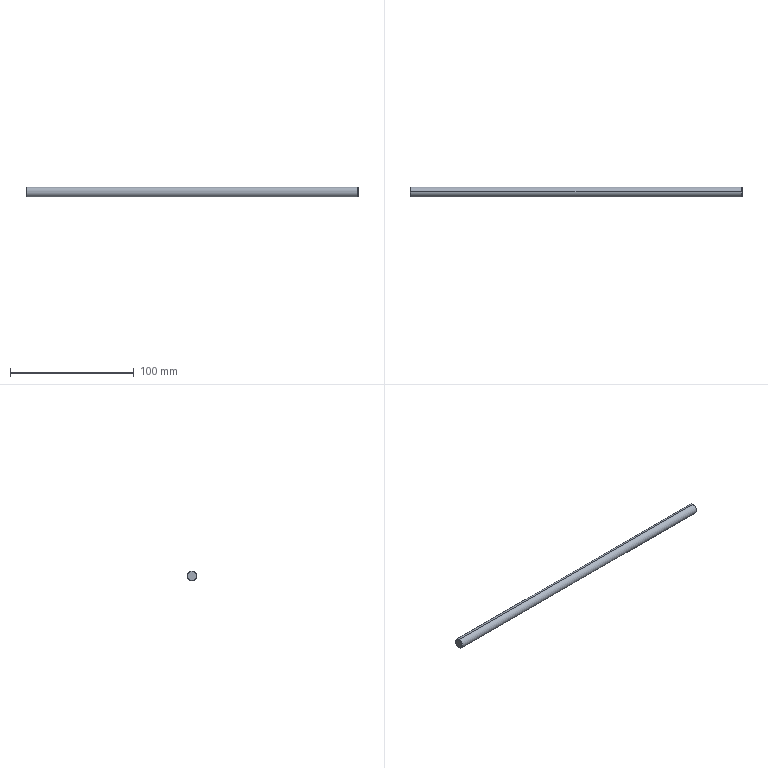Component | SolidWorks | STB-08-010-1 | 1 solid | 8 faces | box 268 x 8 x 8 mm | volume 13465 mm3 | cone 4 | cylinder 2 | plane 2 | commonest cylinder face diameters 8 x2
build123d program:
from build123d import *

# Parameters (mm, degrees)
SKETCH1_R           = 4
BOSS_EXTRUDE1_DEPTH = 134
CHAMFER1_SIZE       = 0.5


with BuildPart() as part:
    # Sketch1 → Boss-Extrude1 (new, symmetric)
    with BuildSketch(Plane(origin=(0, 0, 0), x_dir=(0, 0, -1), z_dir=(1, 0, 0))):
        Circle(SKETCH1_R)
    extrude(amount=BOSS_EXTRUDE1_DEPTH, both=True)

    # Chamfer1
    chamfer1_edges = [part.edges().sort_by_distance(p)[0] for p in [
        (-134, 0, 4),
        (134, 0, 4),
    ]]
    chamfer(chamfer1_edges, length=CHAMFER1_SIZE)


solid = part.part

# Placed as in the assembly
solid = solid.moved(Location((-104.904, 65.999, -19), (0, 0, 0)))
STEP:
#1=CARTESIAN_POINT('',(1.146,2.598,-0.8858));
#2=VERTEX_POINT('',#1);
#3=CARTESIAN_POINT('',(1.146,2.598,-0.6102));
#4=VERTEX_POINT('',#3);
#5=CARTESIAN_POINT('',(1.146,2.598,-0.748));
#6=DIRECTION('',(1.,0.,0.));
#7=DIRECTION('',(0.,0.,-1.));
#8=AXIS2_PLACEMENT_3D('',#5,#6,#7);
#9=CIRCLE('',#8,0.1378);
#10=EDGE_CURVE('',#2,#4,#9,.T.);
#11=ORIENTED_EDGE('',*,*,#10,.F.);
#12=CARTESIAN_POINT('',(1.126,2.598,-0.9055));
#13=VERTEX_POINT('',#12);
#14=CARTESIAN_POINT('',(1.146,2.598,-0.8858));
#15=DIRECTION('',(-0.7071,0.,-0.7071));
#16=VECTOR('',#15,39.37);
#17=LINE('',#14,#16);
#18=EDGE_CURVE('',#2,#13,#17,.T.);
#19=ORIENTED_EDGE('',*,*,#18,.T.);
#20=CARTESIAN_POINT('',(1.126,2.598,-0.5906));
#21=VERTEX_POINT('',#20);
#22=CARTESIAN_POINT('',(1.126,2.598,-0.748));
#23=DIRECTION('',(-1.,0.,0.));
#24=DIRECTION('',(0.,0.,-1.));
#25=AXIS2_PLACEMENT_3D('',#22,#23,#24);
#26=CIRCLE('',#25,0.1575);
#27=EDGE_CURVE('',#21,#13,#26,.T.);
#28=ORIENTED_EDGE('',*,*,#27,.F.);
#29=CARTESIAN_POINT('',(1.146,2.598,-0.6102));
#30=DIRECTION('',(-0.7071,0.,0.7071));
#31=VECTOR('',#30,39.37);
#32=LINE('',#29,#31);
#33=EDGE_CURVE('',#4,#21,#32,.T.);
#34=ORIENTED_EDGE('',*,*,#33,.F.);
#35=EDGE_LOOP('',(#11,#19,#28,#34));
#36=FACE_OUTER_BOUND('',#35,.T.);
#37=CARTESIAN_POINT('',(1.146,2.598,-0.748));
#38=DIRECTION('',(-1.,0.,0.));
#39=DIRECTION('',(0.,0.,1.));
#40=AXIS2_PLACEMENT_3D('',#37,#38,#39);
#41=CONICAL_SURFACE('',#40,0.1378,0.7854);
#42=ADVANCED_FACE('',(#36),#41,.T.);
#43=CARTESIAN_POINT('',(-9.406,2.598,-0.6102));
#44=VERTEX_POINT('',#43);
#45=CARTESIAN_POINT('',(-9.406,2.598,-0.8858));
#46=VERTEX_POINT('',#45);
#47=CARTESIAN_POINT('',(-9.406,2.598,-0.748));
#48=DIRECTION('',(-1.,0.,0.));
#49=DIRECTION('',(0.,0.,-1.));
#50=AXIS2_PLACEMENT_3D('',#47,#48,#49);
#51=CIRCLE('',#50,0.1378);
#52=EDGE_CURVE('',#44,#46,#51,.T.);
#53=ORIENTED_EDGE('',*,*,#52,.F.);
#54=CARTESIAN_POINT('',(-9.386,2.598,-0.5906));
#55=VERTEX_POINT('',#54);
#56=CARTESIAN_POINT('',(-9.386,2.598,-0.5906));
#57=DIRECTION('',(0.7071,0.,0.7071));
#58=VECTOR('',#57,39.37);
#59=LINE('',#56,#58);
#60=EDGE_CURVE('',#44,#55,#59,.T.);
#61=ORIENTED_EDGE('',*,*,#60,.T.);
#62=CARTESIAN_POINT('',(-9.386,2.598,-0.9055));
#63=VERTEX_POINT('',#62);
#64=CARTESIAN_POINT('',(-9.386,2.598,-0.748));
#65=DIRECTION('',(1.,0.,0.));
#66=DIRECTION('',(0.,0.,-1.));
#67=AXIS2_PLACEMENT_3D('',#64,#65,#66);
#68=CIRCLE('',#67,0.1575);
#69=EDGE_CURVE('',#63,#55,#68,.T.);
#70=ORIENTED_EDGE('',*,*,#69,.F.);
#71=CARTESIAN_POINT('',(-9.386,2.598,-0.9055));
#72=DIRECTION('',(0.7071,0.,-0.7071));
#73=VECTOR('',#72,39.37);
#74=LINE('',#71,#73);
#75=EDGE_CURVE('',#46,#63,#74,.T.);
#76=ORIENTED_EDGE('',*,*,#75,.F.);
#77=EDGE_LOOP('',(#53,#61,#70,#76));
#78=FACE_OUTER_BOUND('',#77,.T.);
#79=CARTESIAN_POINT('',(-9.386,2.598,-0.748));
#80=DIRECTION('',(1.,0.,0.));
#81=DIRECTION('',(0.,0.,-1.));
#82=AXIS2_PLACEMENT_3D('',#79,#80,#81);
#83=CONICAL_SURFACE('',#82,0.1575,0.7854);
#84=ADVANCED_FACE('',(#78),#83,.T.);
#85=ORIENTED_EDGE('',*,*,#27,.T.);
#86=CARTESIAN_POINT('',(1.146,2.598,-0.9055));
#87=DIRECTION('',(-1.,0.,0.));
#88=VECTOR('',#87,39.37);
#89=LINE('',#86,#88);
#90=EDGE_CURVE('',#13,#63,#89,.T.);
#91=ORIENTED_EDGE('',*,*,#90,.T.);
#92=ORIENTED_EDGE('',*,*,#69,.T.);
#93=CARTESIAN_POINT('',(1.146,2.598,-0.5906));
#94=DIRECTION('',(-1.,0.,0.));
#95=VECTOR('',#94,39.37);
#96=LINE('',#93,#95);
#97=EDGE_CURVE('',#21,#55,#96,.T.);
#98=ORIENTED_EDGE('',*,*,#97,.F.);
#99=EDGE_LOOP('',(#85,#91,#92,#98));
#100=FACE_OUTER_BOUND('',#99,.T.);
#101=CARTESIAN_POINT('',(1.146,2.598,-0.748));
#102=DIRECTION('',(-1.,0.,0.));
#103=DIRECTION('',(0.,0.,1.));
#104=AXIS2_PLACEMENT_3D('',#101,#102,#103);
#105=CYLINDRICAL_SURFACE('',#104,0.1575);
#106=ADVANCED_FACE('',(#100),#105,.T.);
#107=ORIENTED_EDGE('',*,*,#90,.F.);
#108=CARTESIAN_POINT('',(1.126,2.598,-0.748));
#109=DIRECTION('',(-1.,0.,0.));
#110=DIRECTION('',(0.,0.,-1.));
#111=AXIS2_PLACEMENT_3D('',#108,#109,#110);
#112=CIRCLE('',#111,0.1575);
#113=EDGE_CURVE('',#13,#21,#112,.T.);
#114=ORIENTED_EDGE('',*,*,#113,.T.);
#115=ORIENTED_EDGE('',*,*,#97,.T.);
#116=CARTESIAN_POINT('',(-9.386,2.598,-0.748));
#117=DIRECTION('',(1.,0.,0.));
#118=DIRECTION('',(0.,0.,-1.));
#119=AXIS2_PLACEMENT_3D('',#116,#117,#118);
#120=CIRCLE('',#119,0.1575);
#121=EDGE_CURVE('',#55,#63,#120,.T.);
#122=ORIENTED_EDGE('',*,*,#121,.T.);
#123=EDGE_LOOP('',(#107,#114,#115,#122));
#124=FACE_OUTER_BOUND('',#123,.T.);
#125=CARTESIAN_POINT('',(1.146,2.598,-0.748));
#126=DIRECTION('',(-1.,0.,0.));
#127=DIRECTION('',(0.,0.,1.));
#128=AXIS2_PLACEMENT_3D('',#125,#126,#127);
#129=CYLINDRICAL_SURFACE('',#128,0.1575);
#130=ADVANCED_FACE('',(#124),#129,.T.);
#131=CARTESIAN_POINT('',(1.146,2.598,-0.748));
#132=DIRECTION('',(1.,0.,0.));
#133=DIRECTION('',(0.,0.,-1.));
#134=AXIS2_PLACEMENT_3D('',#131,#132,#133);
#135=CIRCLE('',#134,0.1378);
#136=EDGE_CURVE('',#4,#2,#135,.T.);
#137=ORIENTED_EDGE('',*,*,#136,.T.);
#138=ORIENTED_EDGE('',*,*,#10,.T.);
#139=EDGE_LOOP('',(#137,#138));
#140=FACE_OUTER_BOUND('',#139,.T.);
#141=CARTESIAN_POINT('',(1.146,2.598,-0.748));
#142=DIRECTION('',(1.,0.,0.));
#143=DIRECTION('',(0.,0.,-1.));
#144=AXIS2_PLACEMENT_3D('',#141,#142,#143);
#145=PLANE('',#144);
#146=ADVANCED_FACE('',(#140),#145,.T.);
#147=CARTESIAN_POINT('',(-9.406,2.598,-0.748));
#148=DIRECTION('',(-1.,0.,0.));
#149=DIRECTION('',(0.,0.,-1.));
#150=AXIS2_PLACEMENT_3D('',#147,#148,#149);
#151=CIRCLE('',#150,0.1378);
#152=EDGE_CURVE('',#46,#44,#151,.T.);
#153=ORIENTED_EDGE('',*,*,#152,.T.);
#154=ORIENTED_EDGE('',*,*,#52,.T.);
#155=EDGE_LOOP('',(#153,#154));
#156=FACE_OUTER_BOUND('',#155,.T.);
#157=CARTESIAN_POINT('',(-9.406,2.598,-0.748));
#158=DIRECTION('',(1.,0.,0.));
#159=DIRECTION('',(0.,0.,-1.));
#160=AXIS2_PLACEMENT_3D('',#157,#158,#159);
#161=PLANE('',#160);
#162=ADVANCED_FACE('',(#156),#161,.F.);
#163=ORIENTED_EDGE('',*,*,#60,.F.);
#164=ORIENTED_EDGE('',*,*,#152,.F.);
#165=ORIENTED_EDGE('',*,*,#75,.T.);
#166=ORIENTED_EDGE('',*,*,#121,.F.);
#167=EDGE_LOOP('',(#163,#164,#165,#166));
#168=FACE_OUTER_BOUND('',#167,.T.);
#169=CARTESIAN_POINT('',(-9.386,2.598,-0.748));
#170=DIRECTION('',(1.,0.,0.));
#171=DIRECTION('',(0.,0.,-1.));
#172=AXIS2_PLACEMENT_3D('',#169,#170,#171);
#173=CONICAL_SURFACE('',#172,0.1575,0.7854);
#174=ADVANCED_FACE('',(#168),#173,.T.);
#175=ORIENTED_EDGE('',*,*,#18,.F.);
#176=ORIENTED_EDGE('',*,*,#136,.F.);
#177=ORIENTED_EDGE('',*,*,#33,.T.);
#178=ORIENTED_EDGE('',*,*,#113,.F.);
#179=EDGE_LOOP('',(#175,#176,#177,#178));
#180=FACE_OUTER_BOUND('',#179,.T.);
#181=CARTESIAN_POINT('',(1.146,2.598,-0.748));
#182=DIRECTION('',(-1.,0.,0.));
#183=DIRECTION('',(0.,0.,1.));
#184=AXIS2_PLACEMENT_3D('',#181,#182,#183);
#185=CONICAL_SURFACE('',#184,0.1378,0.7854);
#186=ADVANCED_FACE('',(#180),#185,.T.);
#187=CLOSED_SHELL('',(#42,#84,#106,#130,#146,#162,#174,#186));
#188=MANIFOLD_SOLID_BREP('',#187);
#189=CARTESIAN_POINT('',(0.,0.,0.));
#190=DIRECTION('',(0.,0.,1.));
#191=DIRECTION('',(1.,0.,0.));
#192=AXIS2_PLACEMENT_3D('',#189,#190,#191);
#193=(LENGTH_UNIT()NAMED_UNIT(*)SI_UNIT($,.METRE.));
#194=LENGTH_MEASURE_WITH_UNIT(LENGTH_MEASURE(0.0254),#193);
#195=DIMENSIONAL_EXPONENTS(1.,0.,0.,0.,0.,0.,0.);
#196=(CONVERSION_BASED_UNIT('',#194)LENGTH_UNIT()NAMED_UNIT(#195));
#197=UNCERTAINTY_MEASURE_WITH_UNIT(LENGTH_MEASURE(0.00001),#196,'','');
#198=(NAMED_UNIT(*)PLANE_ANGLE_UNIT()SI_UNIT($,.RADIAN.));
#199=(NAMED_UNIT(*)SI_UNIT($,.STERADIAN.)SOLID_ANGLE_UNIT());
#200=(GEOMETRIC_REPRESENTATION_CONTEXT(3)GLOBAL_UNCERTAINTY_ASSIGNED_CONTEXT((#197))GLOBAL_UNIT_ASSIGNED_CONTEXT((#196,#198,#199))REPRESENTATION_CONTEXT('',''));
#201=ADVANCED_BREP_SHAPE_REPRESENTATION('',(#188,#192),#200);
#202=COLOUR_RGB('',0.7922,0.8196,0.9333);
#203=FILL_AREA_STYLE_COLOUR('',#202);
#204=FILL_AREA_STYLE('',(#203));
#205=SURFACE_STYLE_FILL_AREA(#204);
#206=SURFACE_SIDE_STYLE('',(#205));
#207=SURFACE_STYLE_USAGE(.BOTH.,#206);
#208=PRESENTATION_STYLE_ASSIGNMENT((#207));
#209=STYLED_ITEM('',(#208),#188);
#210=(LENGTH_UNIT()NAMED_UNIT(*)SI_UNIT($,.METRE.));
#211=LENGTH_MEASURE_WITH_UNIT(LENGTH_MEASURE(0.0254),#210);
#212=DIMENSIONAL_EXPONENTS(1.,0.,0.,0.,0.,0.,0.);
#213=(CONVERSION_BASED_UNIT('',#211)LENGTH_UNIT()NAMED_UNIT(#212));
#214=UNCERTAINTY_MEASURE_WITH_UNIT(LENGTH_MEASURE(0.00001),#213,'','');
#215=(NAMED_UNIT(*)PLANE_ANGLE_UNIT()SI_UNIT($,.RADIAN.));
#216=(NAMED_UNIT(*)SI_UNIT($,.STERADIAN.)SOLID_ANGLE_UNIT());
#217=(GEOMETRIC_REPRESENTATION_CONTEXT(3)GLOBAL_UNCERTAINTY_ASSIGNED_CONTEXT((#214))GLOBAL_UNIT_ASSIGNED_CONTEXT((#213,#215,#216))REPRESENTATION_CONTEXT('',''));
#218=MECHANICAL_DESIGN_GEOMETRIC_PRESENTATION_REPRESENTATION('',(#209),#217);
#219=PRESENTATION_LAYER_ASSIGNMENT('','',(#209));